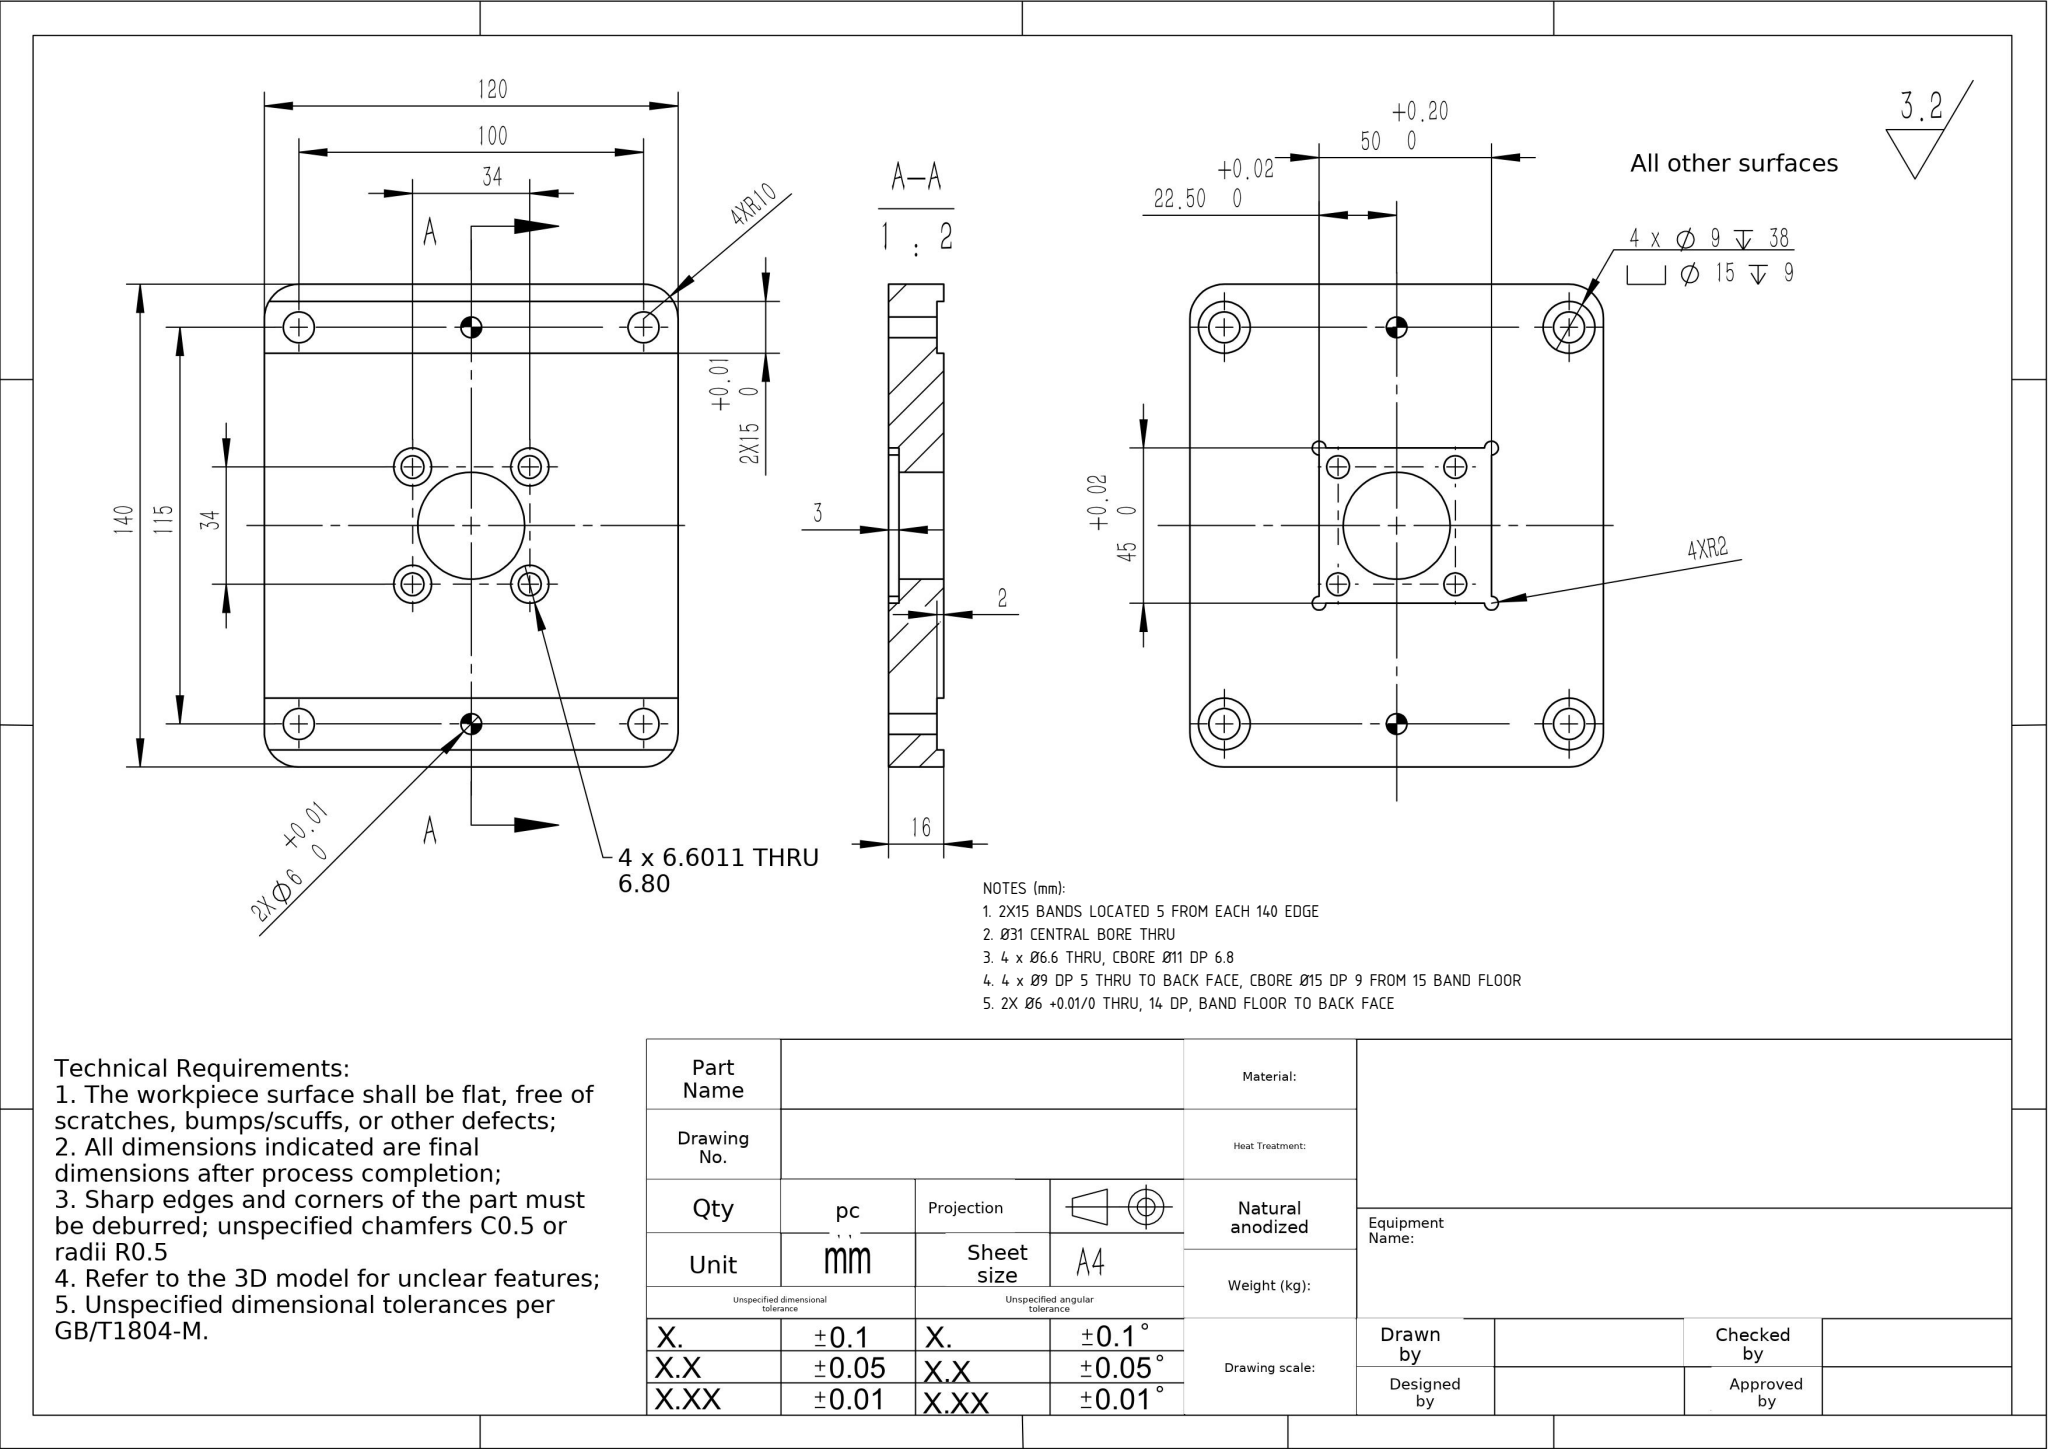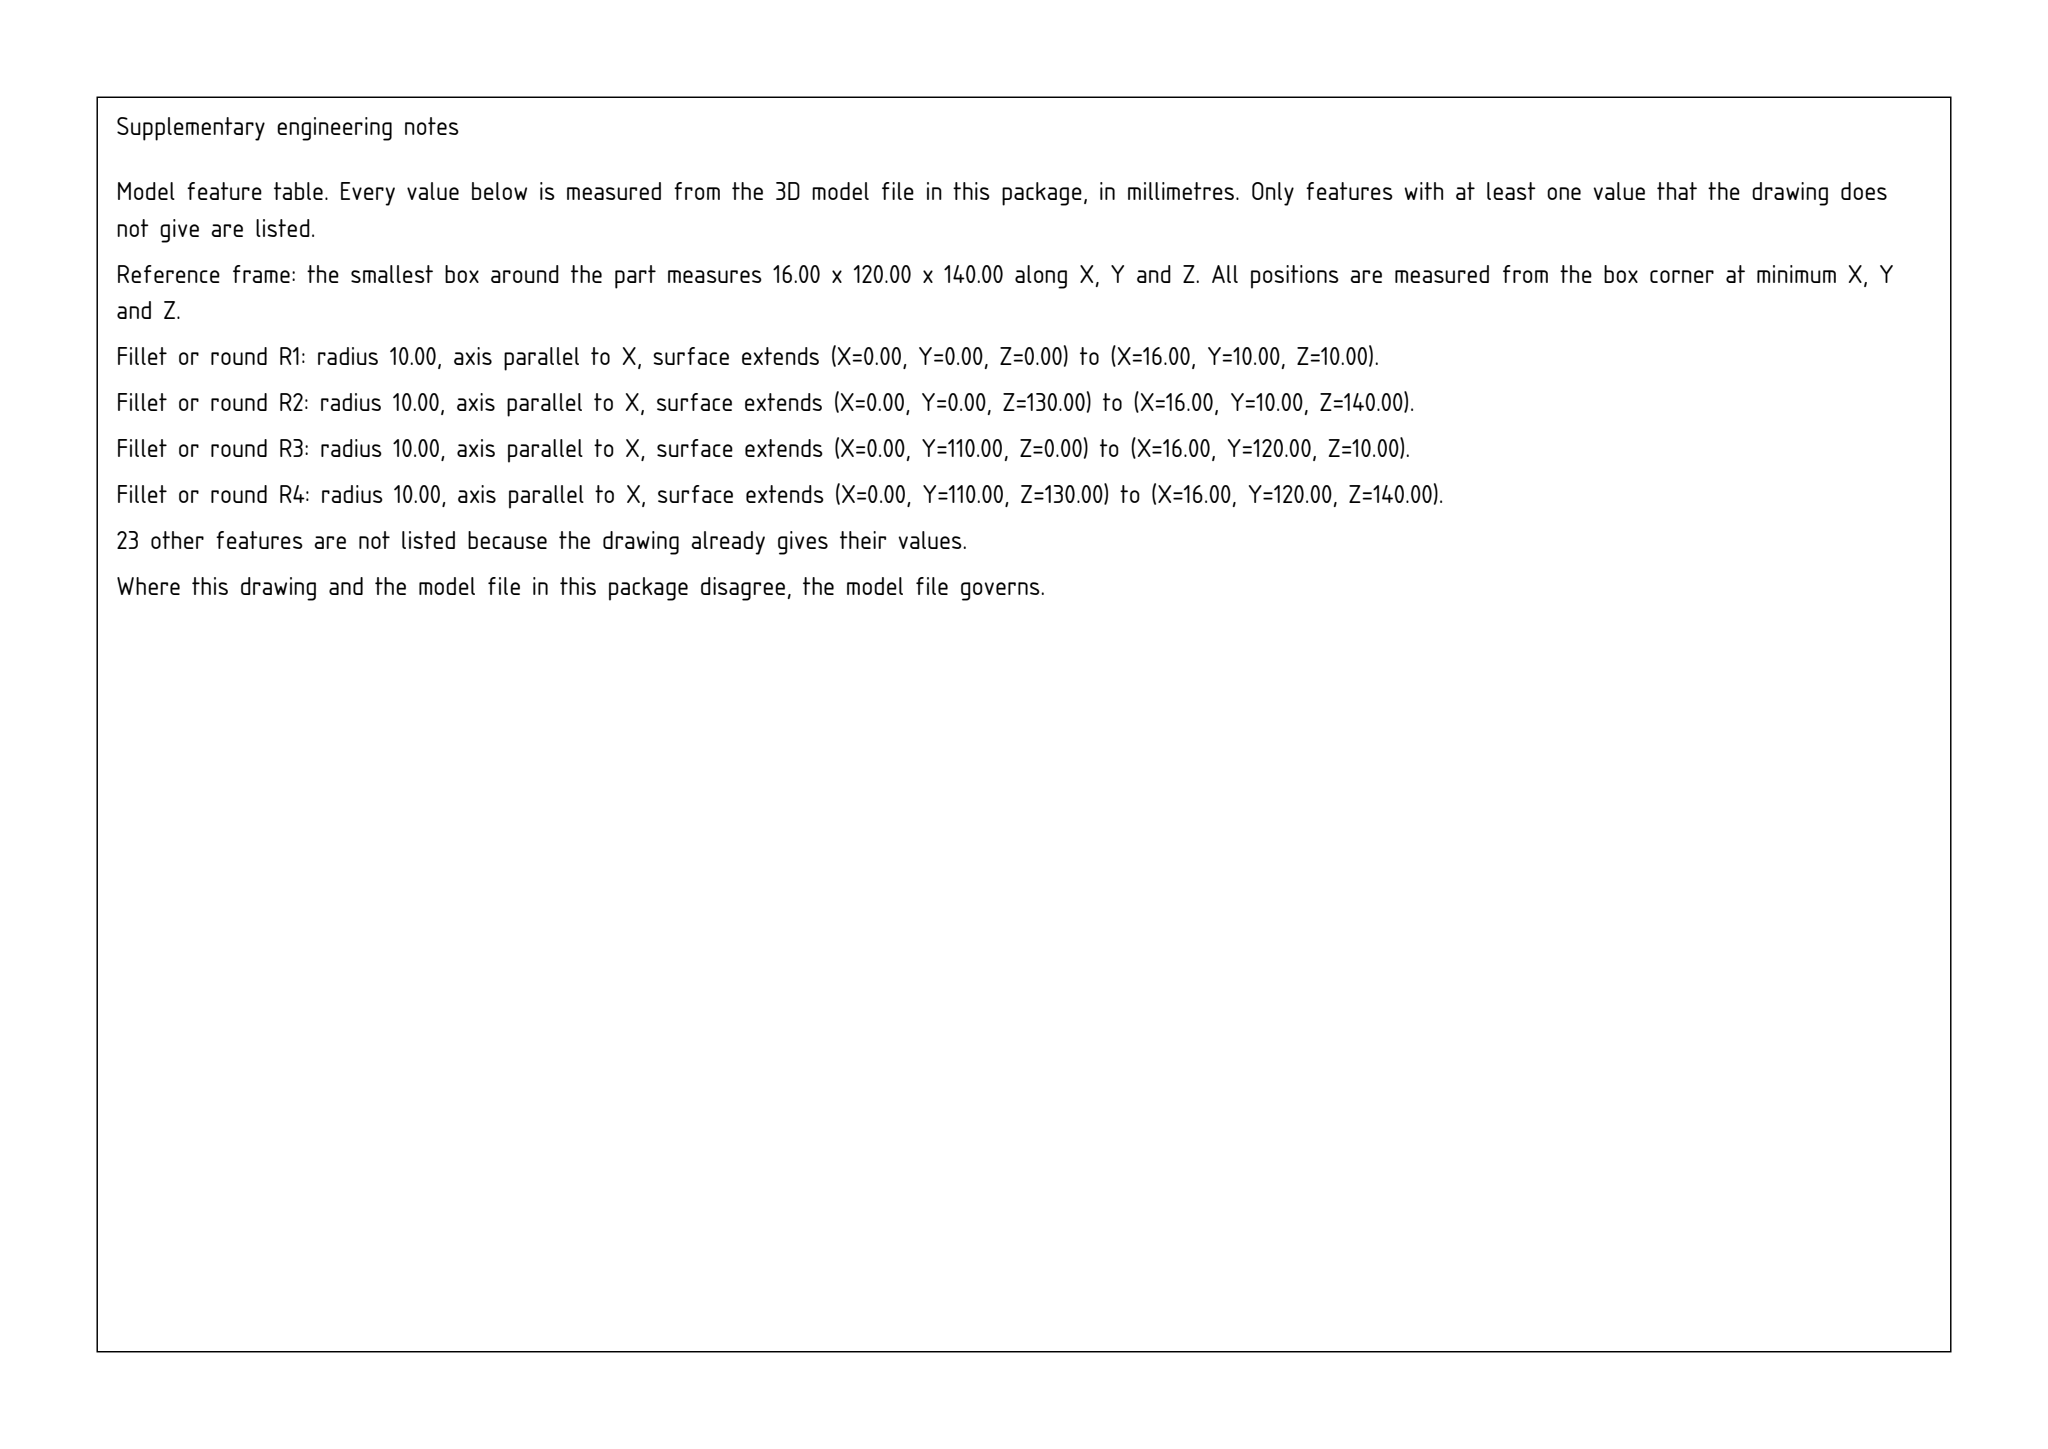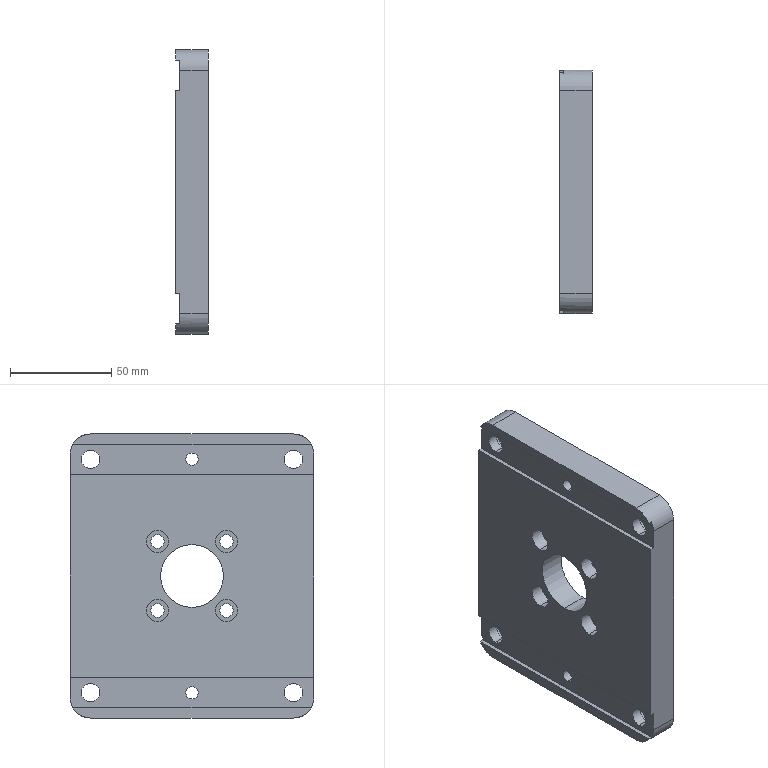Part | SolidWorks | mm | 1 solid | 75 faces | box 16 x 120 x 140 mm | volume 231710 mm3 | cylinder 48 | plane 27 | commonest cylinder face diameters 15 x8 9 x8 11 x8 6.6 x8 4 x6 6 x4 20 x4 31 x2
Drawing notes:
2X15 BANDS LOCATED 5 FROM EACH 140 EDGE | from the solid: z planes at 5/20 and 120/135 with bbox z=140; band floors x=2 (count 2)
Ø31 CENTRAL BORE THRU | from the solid: cyl dia 31.0 axis x at y60/z70, len 13.0 meets 3 deep recess = thru 16 plate
4 x Ø6.6 THRU, CBORE Ø11 DP 6.8 | from the solid: cyl 6.6 len 6.2 coaxial with cyl 11.0 len 6.8 at (43,53)(43,87)(77,53)(77,87)
4 x Ø9 DP 5 THRU TO BACK FACE, CBORE Ø15 DP 9 FROM 15 BAND FLOOR | from the solid: Ø9 len 5.0 and Ø15 len 9.0 at (y,z)=(10/110, 12.5/127.5); x planes 2.0->11->16, plate 16 thk
2X Ø6 +0.01/0 THRU, 14 DP, BAND FLOOR TO BACK FACE | from the solid: Ø6 cyl axis x len 14 at (y60,z12.5) and (y60,z127.5); runs x=2 to x=16
build123d program:
from build123d import *

# Parameters (mm, degrees)
SKETCH1_W                                         = 140
SKETCH1_H                                         = 120
BOSS_EXTRUDE1_DEPTH                               = 16
SKETCH2_R                                         = 15.5
CUT_EXTRUDE1_DEPTH                                = 94.574
HOLE_SIZE_ACCORDING_TO_HEXAGON_SOCKET_D           = 6.6
HOLE_SIZE_ACCORDING_TO_HEXAGON_SOCKET_CBORE_D     = 11
HOLE_SIZE_ACCORDING_TO_HEXAGON_SOCKET_CBORE_DEPTH = 6.8
SKETCH9_W                                         = 15
SKETCH9_H                                         = 120
CUT_EXTRUDE3_DEPTH                                = 2
HOLE_SIZE_ACCORDING_TO_HEXAGON_SO_2_D             = 9
HOLE_SIZE_ACCORDING_TO_HEXAGON_SO_2_DEPTH         = 38
HOLE_SIZE_ACCORDING_TO_HEXAGON_SO_2_CBORE_D       = 15
HOLE_SIZE_ACCORDING_TO_HEXAGON_SO_2_CBORE_DEPTH   = 9
HOLE_SIZE_ACCORDING_TO_HEXAGON_SO_2_TIP           = 2.704
FILLET1_R                                         = 10
SIZE_MM_DOWEL_PIN_HOLE1_D                         = 6
CUT_EXTRUDE4_DEPTH                                = 3
SKETCH15_R                                        = 2
CUT_EXTRUDE5_DEPTH                                = 3


with BuildPart() as part:
    # Sketch1 → Boss-Extrude1 (new body)
    with BuildSketch(Plane(origin=(0, 0, 0), x_dir=(0, 0, -1), z_dir=(1, 0, 0))):
        Rectangle(SKETCH1_W, SKETCH1_H)
    extrude(amount=BOSS_EXTRUDE1_DEPTH)

    # Sketch2 → Cut-Extrude1 (cut, through all)
    with BuildSketch(Plane.ZY):
        Circle(SKETCH2_R)
    extrude(amount=-CUT_EXTRUDE1_DEPTH, mode=Mode.SUBTRACT)

    # Hole Size _ according to_ Hexagon Socket (through all)
    with Locations(Plane(origin=(0, 17, 17), x_dir=(0, 0, -1), z_dir=(-1, 0, 0))):
        with Locations((0, 0), (34, 0), (34, 34), (0, 34)):
            CounterBoreHole(HOLE_SIZE_ACCORDING_TO_HEXAGON_SOCKET_D / 2, HOLE_SIZE_ACCORDING_TO_HEXAGON_SOCKET_CBORE_D / 2, HOLE_SIZE_ACCORDING_TO_HEXAGON_SOCKET_CBORE_DEPTH)

    # Sketch9 → Cut-Extrude3 (cut)
    with BuildSketch(Plane.ZY):
        with Locations((-57.5, 0)):
            Rectangle(SKETCH9_W, SKETCH9_H)
        with Locations((57.5, 0)):
            Rectangle(SKETCH9_W, SKETCH9_H)
    extrude(amount=-CUT_EXTRUDE3_DEPTH, mode=Mode.SUBTRACT)

    # Hole Size _ according to_ Hexagon So 2
    with Locations(Plane(origin=(16, -50, 57.5), x_dir=(0, 0, 1), z_dir=(1, 0, 0))):
        with Locations((0, 0), (-115, -100), (-115, 0), (0, -100)):
            CounterBoreHole(HOLE_SIZE_ACCORDING_TO_HEXAGON_SO_2_D / 2, HOLE_SIZE_ACCORDING_TO_HEXAGON_SO_2_CBORE_D / 2, HOLE_SIZE_ACCORDING_TO_HEXAGON_SO_2_CBORE_DEPTH, depth=HOLE_SIZE_ACCORDING_TO_HEXAGON_SO_2_DEPTH)
            with Locations((0, 0, -(HOLE_SIZE_ACCORDING_TO_HEXAGON_SO_2_DEPTH + HOLE_SIZE_ACCORDING_TO_HEXAGON_SO_2_TIP / 2))):  # 118° drill point
                Cone(0, HOLE_SIZE_ACCORDING_TO_HEXAGON_SO_2_D / 2, HOLE_SIZE_ACCORDING_TO_HEXAGON_SO_2_TIP, mode=Mode.SUBTRACT)

    # Fillet1
    fillet1_edges = [part.edges().sort_by_distance(p)[0] for p in [
        (8, 60, 70),
        (8, 60, -70),
        (8, -60, -70),
        (8, -60, 70),
    ]]
    fillet(fillet1_edges, radius=FILLET1_R)

    # Size mm Dowel Pin Hole1 (through all)
    with Locations(Plane(origin=(16, 0, 57.5), x_dir=(0, 0, 1), z_dir=(1, 0, 0))):
        with Locations((0, 0), (-115, 0)):
            Hole(SIZE_MM_DOWEL_PIN_HOLE1_D / 2)

    # Sketch14 → Cut-Extrude4 (cut)
    with BuildSketch(Plane(origin=(16, 0, 0), x_dir=(0, 0, -1), z_dir=(1, 0, 0))):
        Polygon((-22.5, 27.5), (22.5, 27.5), (22.5, 22.5), (22.5, -22.5), (-22.5, -22.5), (-22.5, 22.5), align=None)
    extrude(amount=-CUT_EXTRUDE4_DEPTH, mode=Mode.SUBTRACT)

    # Sketch15 → Cut-Extrude5 (cut)
    with BuildSketch(Plane(origin=(16, 0, 0), x_dir=(0, 0, -1), z_dir=(1, 0, 0))):
        with Locations((-22.5, 27.5)):
            Circle(SKETCH15_R)
        with Locations((22.5, 27.5)):
            Circle(SKETCH15_R)
        with Locations((22.5, -22.5)):
            Circle(SKETCH15_R)
        with Locations((-22.5, -22.5)):
            Circle(SKETCH15_R)
    extrude(amount=-CUT_EXTRUDE5_DEPTH, mode=Mode.SUBTRACT)


solid = part.part